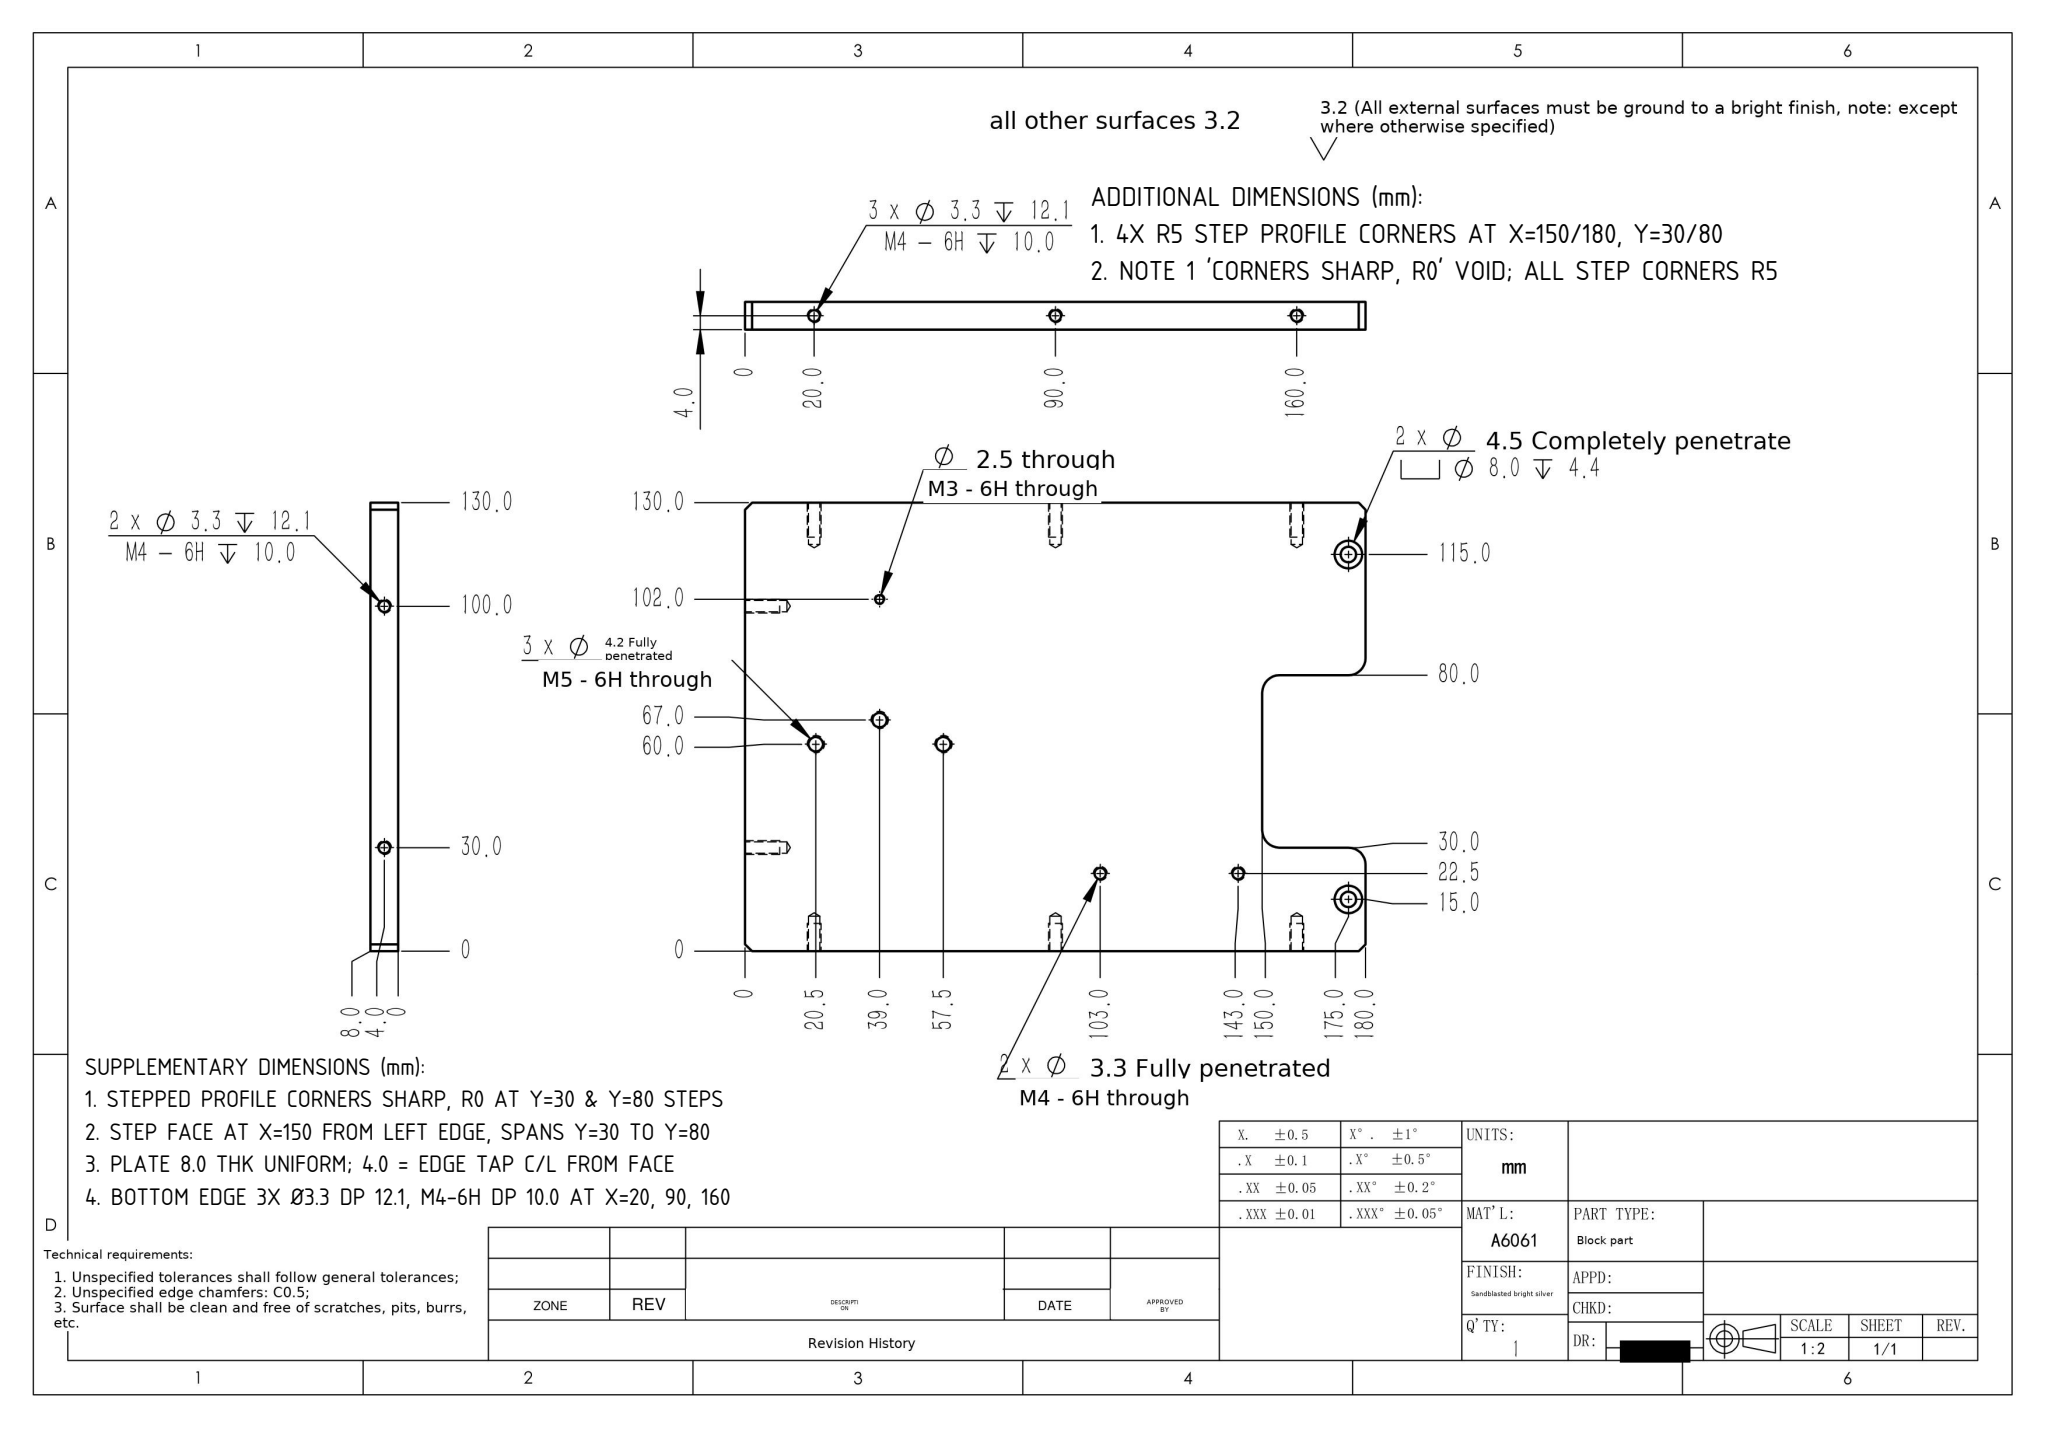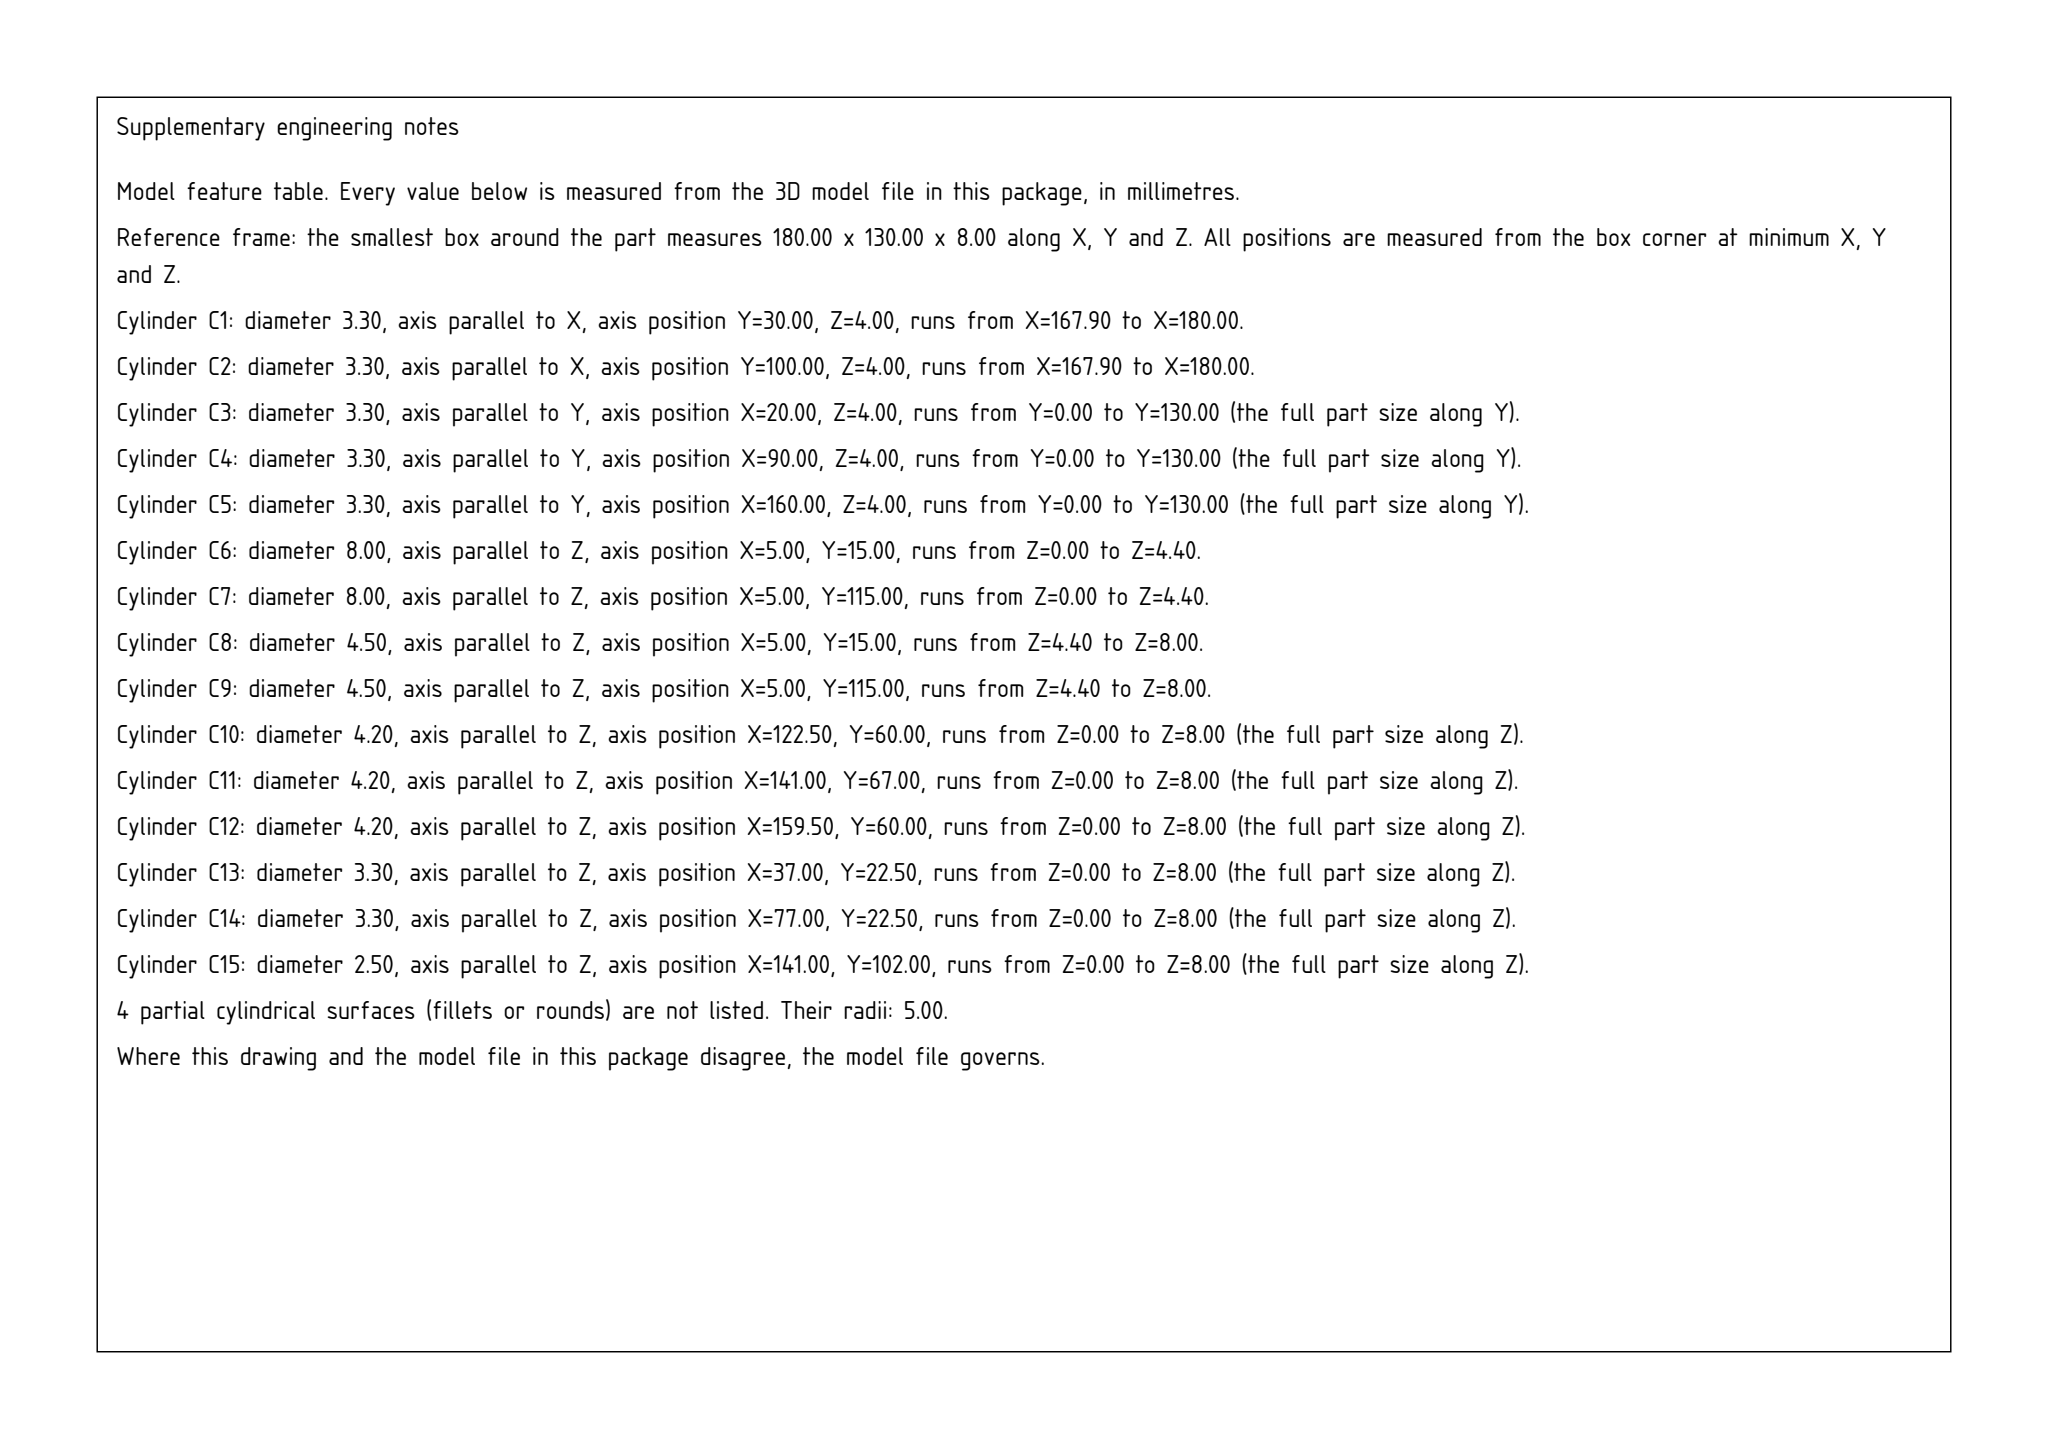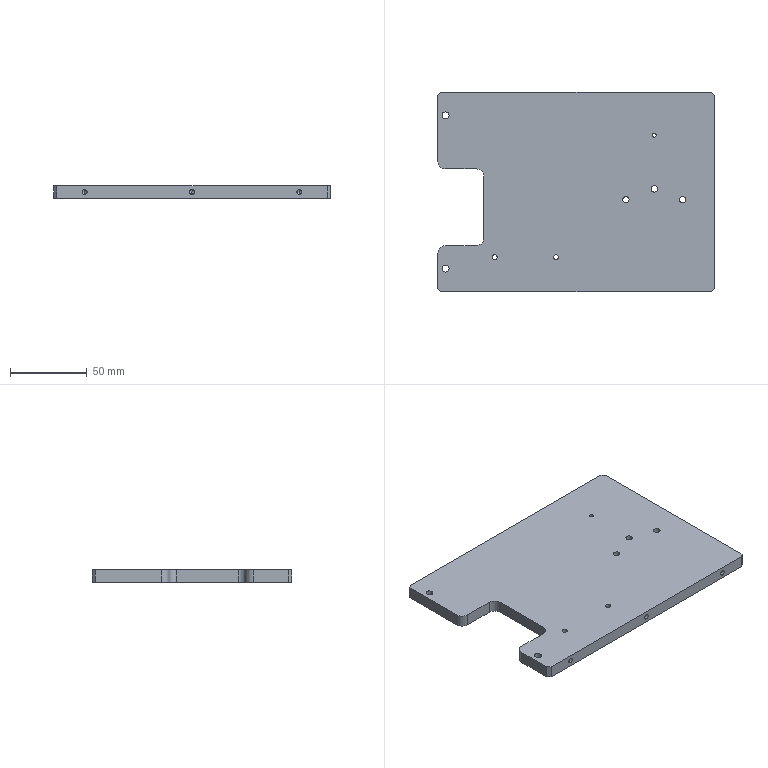Part | SolidWorks | mm | 1 solid | 72 faces | box 180 x 130 x 8 mm | volume 173271 mm3 | cylinder 40 | cone 16 | plane 16 | commonest cylinder face diameters 3.3 x20 4.2 x6 8 x4 4.5 x4 10 x4 2.5 x2
build123d program:
from build123d import *

# Parameters (mm, degrees)
SKETCH1_W                                       = 180
SKETCH1_H                                       = 130
BOSS_EXTRUDE1_DEPTH                             = 8
M4_HEX_SOCKET_HEAD_CAP_SCREW_CBORE1_D           = 4.5
M4_HEX_SOCKET_HEAD_CAP_SCREW_CBORE1_CBORE_D     = 8
M4_HEX_SOCKET_HEAD_CAP_SCREW_CBORE1_CBORE_DEPTH = 4.4
M4_TAPPED_HOLE3_D                               = 3.3
M4_TAPPED_HOLE3_DEPTH                           = 12.1
M4_TAPPED_HOLE3_TIP                             = 0.9914
M4_TAPPED_HOLE1_D                               = 3.3
M4_TAPPED_HOLE4_D                               = 3.3
M4_TAPPED_HOLE4_DEPTH                           = 10.1
M4_TAPPED_HOLE4_TIP                             = 0.9914
SKETCH17_W                                      = 30
SKETCH17_H                                      = 50
CUT_EXTRUDE1_DEPTH                              = 112.306
M5_TAPPED_HOLE1_D                               = 4.2
M3_TAPPED_HOLE3_D                               = 2.5
M4_TAPPED_HOLE2_D                               = 3.3
M4_TAPPED_HOLE2_DEPTH                           = 12.1
M4_TAPPED_HOLE2_TIP                             = 0.9914
CHAMFER1_SIZE                                   = 2
FILLET1_R                                       = 5


with BuildPart() as part:
    # Sketch1 → Boss-Extrude1 (new body)
    with BuildSketch(Plane.XY):
        Rectangle(SKETCH1_W, SKETCH1_H)
    extrude(amount=BOSS_EXTRUDE1_DEPTH)

    # M4 Hex Socket Head Cap Screw CBORE1 (through all)
    with Locations(Plane(origin=(0, 0, 0), x_dir=(-1, 0, 0), z_dir=(0, 0, -1))):
        with Locations((85, 50), (85, -50)):
            CounterBoreHole(M4_HEX_SOCKET_HEAD_CAP_SCREW_CBORE1_D / 2, M4_HEX_SOCKET_HEAD_CAP_SCREW_CBORE1_CBORE_D / 2, M4_HEX_SOCKET_HEAD_CAP_SCREW_CBORE1_CBORE_DEPTH)

    # M4 Tapped Hole3
    with Locations(Plane(origin=(0, 65, 0), x_dir=(1, 0, 0), z_dir=(0, 1, 0))):
        with Locations((-70, -4), (0, -4), (70, -4)):
            Hole(M4_TAPPED_HOLE3_D / 2, depth=M4_TAPPED_HOLE3_DEPTH)
            with Locations((0, 0, -(M4_TAPPED_HOLE3_DEPTH + M4_TAPPED_HOLE3_TIP / 2))):  # 118° drill point
                Cone(0, M4_TAPPED_HOLE3_D / 2, M4_TAPPED_HOLE3_TIP, mode=Mode.SUBTRACT)

    # M4 Tapped Hole1 (through all)
    with Locations(Plane(origin=(0, 0, 0), x_dir=(-1, 0, 0), z_dir=(0, 0, -1))):
        with Locations((53, -42.5), (13, -42.5)):
            Hole(M4_TAPPED_HOLE1_D / 2)

    # M4 Tapped Hole4
    with Locations(Plane(origin=(0, -65, 0), x_dir=(-1, 0, 0), z_dir=(0, -1, 0))):
        with Locations((-70, -4), (0, -4), (70, -4)):
            Hole(M4_TAPPED_HOLE4_D / 2, depth=M4_TAPPED_HOLE4_DEPTH)
            with Locations((0, 0, -(M4_TAPPED_HOLE4_DEPTH + M4_TAPPED_HOLE4_TIP / 2))):  # 118° drill point
                Cone(0, M4_TAPPED_HOLE4_D / 2, M4_TAPPED_HOLE4_TIP, mode=Mode.SUBTRACT)

    # Sketch17 → Cut-Extrude1 (cut, through all)
    with BuildSketch(Plane(origin=(0, 0, 0), x_dir=(-1, 0, 0), z_dir=(0, 0, -1))):
        with Locations((75, -10)):
            Rectangle(SKETCH17_W, SKETCH17_H)
    extrude(amount=-CUT_EXTRUDE1_DEPTH, mode=Mode.SUBTRACT)

    # M5 Tapped Hole1 (through all)
    with Locations(Plane(origin=(0, 0, 0), x_dir=(-1, 0, 0), z_dir=(0, 0, -1))):
        with Locations((-32.5, -5), (-51, 2), (-69.5, -5)):
            Hole(M5_TAPPED_HOLE1_D / 2)

    # M3 Tapped Hole3 (through all)
    with Locations(Plane(origin=(0, 0, 0), x_dir=(-1, 0, 0), z_dir=(0, 0, -1))):
        with Locations((-51, 37)):
            Hole(M3_TAPPED_HOLE3_D / 2)

    # M4 Tapped Hole2
    with Locations(Plane(origin=(90, 0, 0), x_dir=(0, 0, -1), z_dir=(1, 0, 0))):
        with Locations((-4, 35), (-4, -35)):
            Hole(M4_TAPPED_HOLE2_D / 2, depth=M4_TAPPED_HOLE2_DEPTH)
            with Locations((0, 0, -(M4_TAPPED_HOLE2_DEPTH + M4_TAPPED_HOLE2_TIP / 2))):  # 118° drill point
                Cone(0, M4_TAPPED_HOLE2_D / 2, M4_TAPPED_HOLE2_TIP, mode=Mode.SUBTRACT)

    # Chamfer1
    chamfer1_edges = [part.edges().sort_by_distance(p)[0] for p in [
        (90, -65, 4),
        (-90, -65, 4),
        (-90, 65, 4),
        (90, 65, 4),
    ]]
    chamfer(chamfer1_edges, length=CHAMFER1_SIZE)

    # Fillet1
    fillet1_edges = [part.edges().sort_by_distance(p)[0] for p in [
        (-90, 15, 4),
        (-90, -35, 4),
        (-60, -35, 4),
        (-60, 15, 4),
    ]]
    fillet(fillet1_edges, radius=FILLET1_R)


solid = part.part